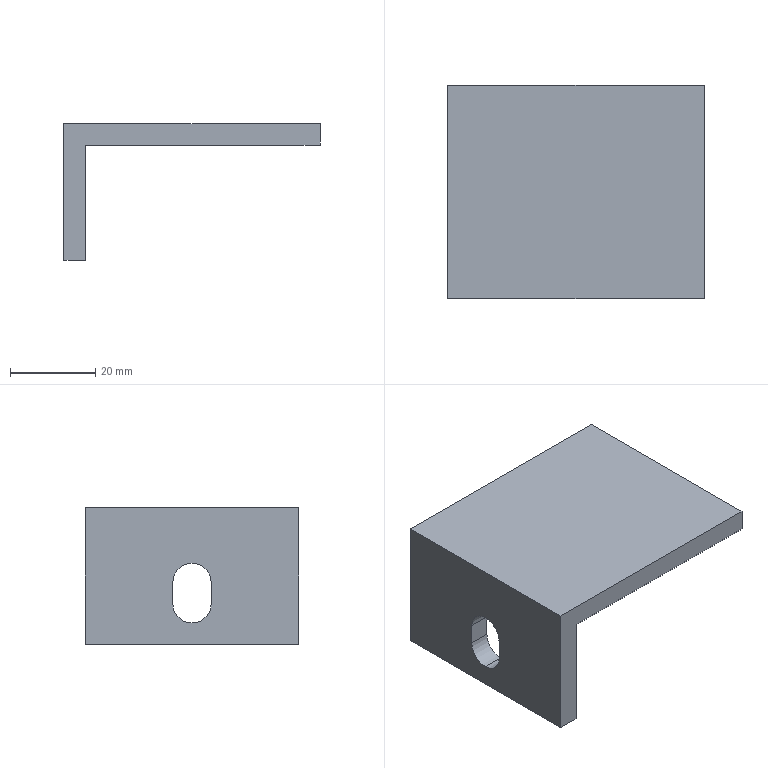Component | SolidWorks | -1-SOLID1-1 | 1 solid | 14 faces | box 60 x 50 x 32 mm | volume 21207 mm3 | plane 10 | cylinder 4 | commonest cylinder face diameters 9 x4
STEP:
#1=CARTESIAN_POINT('',(-15.551,-30.138,50.197));
#2=VERTEX_POINT('',#1);
#3=CARTESIAN_POINT('',(-15.551,-30.315,50.374));
#4=VERTEX_POINT('',#3);
#5=CARTESIAN_POINT('',(-15.551,-30.315,50.197));
#6=DIRECTION('',(1.,0.,-0.));
#7=DIRECTION('',(0.,-1.,0.));
#8=AXIS2_PLACEMENT_3D('',#5,#6,#7);
#9=CIRCLE('',#8,0.1772);
#10=EDGE_CURVE('',#2,#4,#9,.T.);
#11=ORIENTED_EDGE('',*,*,#10,.T.);
#12=CARTESIAN_POINT('',(-15.748,-30.315,50.374));
#13=VERTEX_POINT('',#12);
#14=CARTESIAN_POINT('',(-13.386,-30.315,50.374));
#15=DIRECTION('',(-1.,-0.,0.));
#16=VECTOR('',#15,39.37);
#17=LINE('',#14,#16);
#18=EDGE_CURVE('',#4,#13,#17,.T.);
#19=ORIENTED_EDGE('',*,*,#18,.T.);
#20=CARTESIAN_POINT('',(-15.748,-30.138,50.197));
#21=VERTEX_POINT('',#20);
#22=CARTESIAN_POINT('',(-15.748,-30.315,50.197));
#23=DIRECTION('',(-1.,-0.,0.));
#24=DIRECTION('',(0.,0.,1.));
#25=AXIS2_PLACEMENT_3D('',#22,#23,#24);
#26=CIRCLE('',#25,0.1772);
#27=EDGE_CURVE('',#13,#21,#26,.T.);
#28=ORIENTED_EDGE('',*,*,#27,.T.);
#29=CARTESIAN_POINT('',(-13.386,-30.138,50.197));
#30=DIRECTION('',(-1.,-0.,0.));
#31=VECTOR('',#30,39.37);
#32=LINE('',#29,#31);
#33=EDGE_CURVE('',#2,#21,#32,.T.);
#34=ORIENTED_EDGE('',*,*,#33,.F.);
#35=EDGE_LOOP('',(#11,#19,#28,#34));
#36=FACE_OUTER_BOUND('',#35,.T.);
#37=CARTESIAN_POINT('',(-13.386,-30.315,50.197));
#38=DIRECTION('',(-1.,-0.,0.));
#39=DIRECTION('',(0.,0.,1.));
#40=AXIS2_PLACEMENT_3D('',#37,#38,#39);
#41=CYLINDRICAL_SURFACE('',#40,0.1772);
#42=ADVANCED_FACE('',(#36),#41,.F.);
#43=CARTESIAN_POINT('',(-15.551,-30.492,50.));
#44=VERTEX_POINT('',#43);
#45=CARTESIAN_POINT('',(-15.551,-30.315,49.823));
#46=VERTEX_POINT('',#45);
#47=CARTESIAN_POINT('',(-15.551,-30.315,50.));
#48=DIRECTION('',(1.,0.,-0.));
#49=DIRECTION('',(0.,-1.,0.));
#50=AXIS2_PLACEMENT_3D('',#47,#48,#49);
#51=CIRCLE('',#50,0.1772);
#52=EDGE_CURVE('',#44,#46,#51,.T.);
#53=ORIENTED_EDGE('',*,*,#52,.T.);
#54=CARTESIAN_POINT('',(-15.748,-30.315,49.823));
#55=VERTEX_POINT('',#54);
#56=CARTESIAN_POINT('',(-13.386,-30.315,49.823));
#57=DIRECTION('',(-1.,-0.,0.));
#58=VECTOR('',#57,39.37);
#59=LINE('',#56,#58);
#60=EDGE_CURVE('',#46,#55,#59,.T.);
#61=ORIENTED_EDGE('',*,*,#60,.T.);
#62=CARTESIAN_POINT('',(-15.748,-30.492,50.));
#63=VERTEX_POINT('',#62);
#64=CARTESIAN_POINT('',(-15.748,-30.315,50.));
#65=DIRECTION('',(-1.,-0.,0.));
#66=DIRECTION('',(0.,0.,-1.));
#67=AXIS2_PLACEMENT_3D('',#64,#65,#66);
#68=CIRCLE('',#67,0.1772);
#69=EDGE_CURVE('',#55,#63,#68,.T.);
#70=ORIENTED_EDGE('',*,*,#69,.T.);
#71=CARTESIAN_POINT('',(-13.386,-30.492,50.));
#72=DIRECTION('',(-1.,-0.,0.));
#73=VECTOR('',#72,39.37);
#74=LINE('',#71,#73);
#75=EDGE_CURVE('',#44,#63,#74,.T.);
#76=ORIENTED_EDGE('',*,*,#75,.F.);
#77=EDGE_LOOP('',(#53,#61,#70,#76));
#78=FACE_OUTER_BOUND('',#77,.T.);
#79=CARTESIAN_POINT('',(-13.386,-30.315,50.));
#80=DIRECTION('',(-1.,-0.,0.));
#81=DIRECTION('',(0.,0.,1.));
#82=AXIS2_PLACEMENT_3D('',#79,#80,#81);
#83=CYLINDRICAL_SURFACE('',#82,0.1772);
#84=ADVANCED_FACE('',(#78),#83,.F.);
#85=CARTESIAN_POINT('',(-13.386,-29.331,50.886));
#86=VERTEX_POINT('',#85);
#87=CARTESIAN_POINT('',(-15.748,-29.331,50.886));
#88=VERTEX_POINT('',#87);
#89=CARTESIAN_POINT('',(-13.386,-29.331,50.886));
#90=DIRECTION('',(-1.,-0.,0.));
#91=VECTOR('',#90,39.37);
#92=LINE('',#89,#91);
#93=EDGE_CURVE('',#86,#88,#92,.T.);
#94=ORIENTED_EDGE('',*,*,#93,.T.);
#95=CARTESIAN_POINT('',(-15.748,-31.299,50.886));
#96=VERTEX_POINT('',#95);
#97=CARTESIAN_POINT('',(-15.748,-31.299,50.886));
#98=DIRECTION('',(-0.,1.,0.));
#99=VECTOR('',#98,39.37);
#100=LINE('',#97,#99);
#101=EDGE_CURVE('',#96,#88,#100,.T.);
#102=ORIENTED_EDGE('',*,*,#101,.F.);
#103=CARTESIAN_POINT('',(-13.386,-31.299,50.886));
#104=VERTEX_POINT('',#103);
#105=CARTESIAN_POINT('',(-13.386,-31.299,50.886));
#106=DIRECTION('',(-1.,-0.,0.));
#107=VECTOR('',#106,39.37);
#108=LINE('',#105,#107);
#109=EDGE_CURVE('',#104,#96,#108,.T.);
#110=ORIENTED_EDGE('',*,*,#109,.F.);
#111=CARTESIAN_POINT('',(-13.386,-31.299,50.886));
#112=DIRECTION('',(-0.,1.,0.));
#113=VECTOR('',#112,39.37);
#114=LINE('',#111,#113);
#115=EDGE_CURVE('',#104,#86,#114,.T.);
#116=ORIENTED_EDGE('',*,*,#115,.T.);
#117=EDGE_LOOP('',(#94,#102,#110,#116));
#118=FACE_OUTER_BOUND('',#117,.T.);
#119=CARTESIAN_POINT('',(-13.386,-31.299,50.886));
#120=DIRECTION('',(-0.,-0.,-1.));
#121=DIRECTION('',(0.,-1.,0.));
#122=AXIS2_PLACEMENT_3D('',#119,#120,#121);
#123=PLANE('',#122);
#124=ADVANCED_FACE('',(#118),#123,.F.);
#125=CARTESIAN_POINT('',(-15.748,-30.492,50.197));
#126=VERTEX_POINT('',#125);
#127=CARTESIAN_POINT('',(-15.748,-30.492,50.197));
#128=DIRECTION('',(-0.,-0.,1.));
#129=VECTOR('',#128,39.37);
#130=LINE('',#127,#129);
#131=EDGE_CURVE('',#63,#126,#130,.T.);
#132=ORIENTED_EDGE('',*,*,#131,.F.);
#133=ORIENTED_EDGE('',*,*,#69,.F.);
#134=CARTESIAN_POINT('',(-15.748,-30.138,50.));
#135=VERTEX_POINT('',#134);
#136=CARTESIAN_POINT('',(-15.748,-30.315,50.));
#137=DIRECTION('',(-1.,-0.,0.));
#138=DIRECTION('',(0.,0.,-1.));
#139=AXIS2_PLACEMENT_3D('',#136,#137,#138);
#140=CIRCLE('',#139,0.1772);
#141=EDGE_CURVE('',#135,#55,#140,.T.);
#142=ORIENTED_EDGE('',*,*,#141,.F.);
#143=CARTESIAN_POINT('',(-15.748,-30.138,50.197));
#144=DIRECTION('',(0.,0.,-1.));
#145=VECTOR('',#144,39.37);
#146=LINE('',#143,#145);
#147=EDGE_CURVE('',#21,#135,#146,.T.);
#148=ORIENTED_EDGE('',*,*,#147,.F.);
#149=ORIENTED_EDGE('',*,*,#27,.F.);
#150=CARTESIAN_POINT('',(-15.748,-30.315,50.197));
#151=DIRECTION('',(-1.,-0.,0.));
#152=DIRECTION('',(0.,0.,1.));
#153=AXIS2_PLACEMENT_3D('',#150,#151,#152);
#154=CIRCLE('',#153,0.1772);
#155=EDGE_CURVE('',#126,#13,#154,.T.);
#156=ORIENTED_EDGE('',*,*,#155,.F.);
#157=EDGE_LOOP('',(#132,#133,#142,#148,#149,#156));
#158=FACE_BOUND('',#157,.T.);
#159=CARTESIAN_POINT('',(-15.748,-29.331,49.626));
#160=VERTEX_POINT('',#159);
#161=CARTESIAN_POINT('',(-15.748,-29.331,50.886));
#162=DIRECTION('',(0.,0.,-1.));
#163=VECTOR('',#162,39.37);
#164=LINE('',#161,#163);
#165=EDGE_CURVE('',#88,#160,#164,.T.);
#166=ORIENTED_EDGE('',*,*,#165,.T.);
#167=CARTESIAN_POINT('',(-15.748,-31.299,49.626));
#168=VERTEX_POINT('',#167);
#169=CARTESIAN_POINT('',(-15.748,-31.299,49.626));
#170=DIRECTION('',(-0.,1.,0.));
#171=VECTOR('',#170,39.37);
#172=LINE('',#169,#171);
#173=EDGE_CURVE('',#168,#160,#172,.T.);
#174=ORIENTED_EDGE('',*,*,#173,.F.);
#175=CARTESIAN_POINT('',(-15.748,-31.299,50.886));
#176=DIRECTION('',(0.,0.,-1.));
#177=VECTOR('',#176,39.37);
#178=LINE('',#175,#177);
#179=EDGE_CURVE('',#96,#168,#178,.T.);
#180=ORIENTED_EDGE('',*,*,#179,.F.);
#181=ORIENTED_EDGE('',*,*,#101,.T.);
#182=EDGE_LOOP('',(#166,#174,#180,#181));
#183=FACE_OUTER_BOUND('',#182,.T.);
#184=CARTESIAN_POINT('',(-15.748,-31.299,50.886));
#185=DIRECTION('',(1.,0.,0.));
#186=DIRECTION('',(0.,0.,-1.));
#187=AXIS2_PLACEMENT_3D('',#184,#185,#186);
#188=PLANE('',#187);
#189=ADVANCED_FACE('',(#158,#183),#188,.F.);
#190=CARTESIAN_POINT('',(-15.551,-29.331,49.626));
#191=VERTEX_POINT('',#190);
#192=CARTESIAN_POINT('',(-15.748,-29.331,49.626));
#193=DIRECTION('',(1.,0.,-0.));
#194=VECTOR('',#193,39.37);
#195=LINE('',#192,#194);
#196=EDGE_CURVE('',#160,#191,#195,.T.);
#197=ORIENTED_EDGE('',*,*,#196,.T.);
#198=CARTESIAN_POINT('',(-15.551,-31.299,49.626));
#199=VERTEX_POINT('',#198);
#200=CARTESIAN_POINT('',(-15.551,-31.299,49.626));
#201=DIRECTION('',(-0.,1.,0.));
#202=VECTOR('',#201,39.37);
#203=LINE('',#200,#202);
#204=EDGE_CURVE('',#199,#191,#203,.T.);
#205=ORIENTED_EDGE('',*,*,#204,.F.);
#206=CARTESIAN_POINT('',(-15.748,-31.299,49.626));
#207=DIRECTION('',(1.,0.,-0.));
#208=VECTOR('',#207,39.37);
#209=LINE('',#206,#208);
#210=EDGE_CURVE('',#168,#199,#209,.T.);
#211=ORIENTED_EDGE('',*,*,#210,.F.);
#212=ORIENTED_EDGE('',*,*,#173,.T.);
#213=EDGE_LOOP('',(#197,#205,#211,#212));
#214=FACE_OUTER_BOUND('',#213,.T.);
#215=CARTESIAN_POINT('',(-15.748,-31.299,49.626));
#216=DIRECTION('',(0.,0.,1.));
#217=DIRECTION('',(-0.,1.,0.));
#218=AXIS2_PLACEMENT_3D('',#215,#216,#217);
#219=PLANE('',#218);
#220=ADVANCED_FACE('',(#214),#219,.F.);
#221=CARTESIAN_POINT('',(-15.551,-30.138,50.));
#222=VERTEX_POINT('',#221);
#223=CARTESIAN_POINT('',(-15.551,-30.138,50.197));
#224=DIRECTION('',(0.,0.,1.));
#225=VECTOR('',#224,39.37);
#226=LINE('',#223,#225);
#227=EDGE_CURVE('',#222,#2,#226,.T.);
#228=ORIENTED_EDGE('',*,*,#227,.F.);
#229=CARTESIAN_POINT('',(-15.551,-30.315,50.));
#230=DIRECTION('',(1.,0.,-0.));
#231=DIRECTION('',(0.,-1.,0.));
#232=AXIS2_PLACEMENT_3D('',#229,#230,#231);
#233=CIRCLE('',#232,0.1772);
#234=EDGE_CURVE('',#46,#222,#233,.T.);
#235=ORIENTED_EDGE('',*,*,#234,.F.);
#236=ORIENTED_EDGE('',*,*,#52,.F.);
#237=CARTESIAN_POINT('',(-15.551,-30.492,50.197));
#238=VERTEX_POINT('',#237);
#239=CARTESIAN_POINT('',(-15.551,-30.492,50.197));
#240=DIRECTION('',(-0.,-0.,-1.));
#241=VECTOR('',#240,39.37);
#242=LINE('',#239,#241);
#243=EDGE_CURVE('',#238,#44,#242,.T.);
#244=ORIENTED_EDGE('',*,*,#243,.F.);
#245=CARTESIAN_POINT('',(-15.551,-30.315,50.197));
#246=DIRECTION('',(1.,0.,-0.));
#247=DIRECTION('',(0.,-1.,0.));
#248=AXIS2_PLACEMENT_3D('',#245,#246,#247);
#249=CIRCLE('',#248,0.1772);
#250=EDGE_CURVE('',#4,#238,#249,.T.);
#251=ORIENTED_EDGE('',*,*,#250,.F.);
#252=ORIENTED_EDGE('',*,*,#10,.F.);
#253=EDGE_LOOP('',(#228,#235,#236,#244,#251,#252));
#254=FACE_BOUND('',#253,.T.);
#255=CARTESIAN_POINT('',(-15.551,-29.331,50.689));
#256=VERTEX_POINT('',#255);
#257=CARTESIAN_POINT('',(-15.551,-29.331,49.626));
#258=DIRECTION('',(0.,0.,1.));
#259=VECTOR('',#258,39.37);
#260=LINE('',#257,#259);
#261=EDGE_CURVE('',#191,#256,#260,.T.);
#262=ORIENTED_EDGE('',*,*,#261,.T.);
#263=CARTESIAN_POINT('',(-15.551,-31.299,50.689));
#264=VERTEX_POINT('',#263);
#265=CARTESIAN_POINT('',(-15.551,-31.299,50.689));
#266=DIRECTION('',(-0.,1.,0.));
#267=VECTOR('',#266,39.37);
#268=LINE('',#265,#267);
#269=EDGE_CURVE('',#264,#256,#268,.T.);
#270=ORIENTED_EDGE('',*,*,#269,.F.);
#271=CARTESIAN_POINT('',(-15.551,-31.299,49.626));
#272=DIRECTION('',(0.,0.,1.));
#273=VECTOR('',#272,39.37);
#274=LINE('',#271,#273);
#275=EDGE_CURVE('',#199,#264,#274,.T.);
#276=ORIENTED_EDGE('',*,*,#275,.F.);
#277=ORIENTED_EDGE('',*,*,#204,.T.);
#278=EDGE_LOOP('',(#262,#270,#276,#277));
#279=FACE_OUTER_BOUND('',#278,.T.);
#280=CARTESIAN_POINT('',(-15.551,-31.299,49.626));
#281=DIRECTION('',(-1.,-0.,0.));
#282=DIRECTION('',(-0.,1.,0.));
#283=AXIS2_PLACEMENT_3D('',#280,#281,#282);
#284=PLANE('',#283);
#285=ADVANCED_FACE('',(#254,#279),#284,.F.);
#286=CARTESIAN_POINT('',(-13.386,-29.331,50.689));
#287=VERTEX_POINT('',#286);
#288=CARTESIAN_POINT('',(-15.551,-29.331,50.689));
#289=DIRECTION('',(1.,0.,-0.));
#290=VECTOR('',#289,39.37);
#291=LINE('',#288,#290);
#292=EDGE_CURVE('',#256,#287,#291,.T.);
#293=ORIENTED_EDGE('',*,*,#292,.T.);
#294=CARTESIAN_POINT('',(-13.386,-31.299,50.689));
#295=VERTEX_POINT('',#294);
#296=CARTESIAN_POINT('',(-13.386,-31.299,50.689));
#297=DIRECTION('',(-0.,1.,0.));
#298=VECTOR('',#297,39.37);
#299=LINE('',#296,#298);
#300=EDGE_CURVE('',#295,#287,#299,.T.);
#301=ORIENTED_EDGE('',*,*,#300,.F.);
#302=CARTESIAN_POINT('',(-15.551,-31.299,50.689));
#303=DIRECTION('',(1.,0.,-0.));
#304=VECTOR('',#303,39.37);
#305=LINE('',#302,#304);
#306=EDGE_CURVE('',#264,#295,#305,.T.);
#307=ORIENTED_EDGE('',*,*,#306,.F.);
#308=ORIENTED_EDGE('',*,*,#269,.T.);
#309=EDGE_LOOP('',(#293,#301,#307,#308));
#310=FACE_OUTER_BOUND('',#309,.T.);
#311=CARTESIAN_POINT('',(-15.551,-31.299,50.689));
#312=DIRECTION('',(0.,0.,1.));
#313=DIRECTION('',(-0.,1.,0.));
#314=AXIS2_PLACEMENT_3D('',#311,#312,#313);
#315=PLANE('',#314);
#316=ADVANCED_FACE('',(#310),#315,.F.);
#317=CARTESIAN_POINT('',(-13.386,-29.331,50.689));
#318=DIRECTION('',(0.,0.,1.));
#319=VECTOR('',#318,39.37);
#320=LINE('',#317,#319);
#321=EDGE_CURVE('',#287,#86,#320,.T.);
#322=ORIENTED_EDGE('',*,*,#321,.T.);
#323=ORIENTED_EDGE('',*,*,#115,.F.);
#324=CARTESIAN_POINT('',(-13.386,-31.299,50.689));
#325=DIRECTION('',(0.,0.,1.));
#326=VECTOR('',#325,39.37);
#327=LINE('',#324,#326);
#328=EDGE_CURVE('',#295,#104,#327,.T.);
#329=ORIENTED_EDGE('',*,*,#328,.F.);
#330=ORIENTED_EDGE('',*,*,#300,.T.);
#331=EDGE_LOOP('',(#322,#323,#329,#330));
#332=FACE_OUTER_BOUND('',#331,.T.);
#333=CARTESIAN_POINT('',(-13.386,-31.299,50.689));
#334=DIRECTION('',(-1.,-0.,0.));
#335=DIRECTION('',(-0.,1.,0.));
#336=AXIS2_PLACEMENT_3D('',#333,#334,#335);
#337=PLANE('',#336);
#338=ADVANCED_FACE('',(#332),#337,.F.);
#339=ORIENTED_EDGE('',*,*,#109,.T.);
#340=ORIENTED_EDGE('',*,*,#179,.T.);
#341=ORIENTED_EDGE('',*,*,#210,.T.);
#342=ORIENTED_EDGE('',*,*,#275,.T.);
#343=ORIENTED_EDGE('',*,*,#306,.T.);
#344=ORIENTED_EDGE('',*,*,#328,.T.);
#345=EDGE_LOOP('',(#339,#340,#341,#342,#343,#344));
#346=FACE_OUTER_BOUND('',#345,.T.);
#347=CARTESIAN_POINT('',(-15.748,-31.299,50.886));
#348=DIRECTION('',(0.,-1.,-0.));
#349=DIRECTION('',(-1.,-0.,0.));
#350=AXIS2_PLACEMENT_3D('',#347,#348,#349);
#351=PLANE('',#350);
#352=ADVANCED_FACE('',(#346),#351,.T.);
#353=ORIENTED_EDGE('',*,*,#93,.F.);
#354=ORIENTED_EDGE('',*,*,#321,.F.);
#355=ORIENTED_EDGE('',*,*,#292,.F.);
#356=ORIENTED_EDGE('',*,*,#261,.F.);
#357=ORIENTED_EDGE('',*,*,#196,.F.);
#358=ORIENTED_EDGE('',*,*,#165,.F.);
#359=EDGE_LOOP('',(#353,#354,#355,#356,#357,#358));
#360=FACE_OUTER_BOUND('',#359,.T.);
#361=CARTESIAN_POINT('',(-15.748,-29.331,50.886));
#362=DIRECTION('',(0.,-1.,-0.));
#363=DIRECTION('',(-1.,-0.,0.));
#364=AXIS2_PLACEMENT_3D('',#361,#362,#363);
#365=PLANE('',#364);
#366=ADVANCED_FACE('',(#360),#365,.F.);
#367=ORIENTED_EDGE('',*,*,#60,.F.);
#368=ORIENTED_EDGE('',*,*,#234,.T.);
#369=CARTESIAN_POINT('',(-13.386,-30.138,50.));
#370=DIRECTION('',(-1.,-0.,0.));
#371=VECTOR('',#370,39.37);
#372=LINE('',#369,#371);
#373=EDGE_CURVE('',#222,#135,#372,.T.);
#374=ORIENTED_EDGE('',*,*,#373,.T.);
#375=ORIENTED_EDGE('',*,*,#141,.T.);
#376=EDGE_LOOP('',(#367,#368,#374,#375));
#377=FACE_OUTER_BOUND('',#376,.T.);
#378=CARTESIAN_POINT('',(-13.386,-30.315,50.));
#379=DIRECTION('',(-1.,-0.,0.));
#380=DIRECTION('',(0.,0.,1.));
#381=AXIS2_PLACEMENT_3D('',#378,#379,#380);
#382=CYLINDRICAL_SURFACE('',#381,0.1772);
#383=ADVANCED_FACE('',(#377),#382,.F.);
#384=ORIENTED_EDGE('',*,*,#227,.T.);
#385=ORIENTED_EDGE('',*,*,#33,.T.);
#386=ORIENTED_EDGE('',*,*,#147,.T.);
#387=ORIENTED_EDGE('',*,*,#373,.F.);
#388=EDGE_LOOP('',(#384,#385,#386,#387));
#389=FACE_OUTER_BOUND('',#388,.T.);
#390=CARTESIAN_POINT('',(-13.386,-30.138,50.197));
#391=DIRECTION('',(-0.,1.,0.));
#392=DIRECTION('',(1.,0.,-0.));
#393=AXIS2_PLACEMENT_3D('',#390,#391,#392);
#394=PLANE('',#393);
#395=ADVANCED_FACE('',(#389),#394,.F.);
#396=ORIENTED_EDGE('',*,*,#18,.F.);
#397=ORIENTED_EDGE('',*,*,#250,.T.);
#398=CARTESIAN_POINT('',(-13.386,-30.492,50.197));
#399=DIRECTION('',(-1.,-0.,0.));
#400=VECTOR('',#399,39.37);
#401=LINE('',#398,#400);
#402=EDGE_CURVE('',#238,#126,#401,.T.);
#403=ORIENTED_EDGE('',*,*,#402,.T.);
#404=ORIENTED_EDGE('',*,*,#155,.T.);
#405=EDGE_LOOP('',(#396,#397,#403,#404));
#406=FACE_OUTER_BOUND('',#405,.T.);
#407=CARTESIAN_POINT('',(-13.386,-30.315,50.197));
#408=DIRECTION('',(-1.,-0.,0.));
#409=DIRECTION('',(0.,0.,1.));
#410=AXIS2_PLACEMENT_3D('',#407,#408,#409);
#411=CYLINDRICAL_SURFACE('',#410,0.1772);
#412=ADVANCED_FACE('',(#406),#411,.F.);
#413=ORIENTED_EDGE('',*,*,#243,.T.);
#414=ORIENTED_EDGE('',*,*,#75,.T.);
#415=ORIENTED_EDGE('',*,*,#131,.T.);
#416=ORIENTED_EDGE('',*,*,#402,.F.);
#417=EDGE_LOOP('',(#413,#414,#415,#416));
#418=FACE_OUTER_BOUND('',#417,.T.);
#419=CARTESIAN_POINT('',(-13.386,-30.492,50.197));
#420=DIRECTION('',(0.,-1.,-0.));
#421=DIRECTION('',(-1.,-0.,0.));
#422=AXIS2_PLACEMENT_3D('',#419,#420,#421);
#423=PLANE('',#422);
#424=ADVANCED_FACE('',(#418),#423,.F.);
#425=CLOSED_SHELL('',(#42,#84,#124,#189,#220,#285,#316,#338,#352,#366,#383,#395,#412,#424));
#426=MANIFOLD_SOLID_BREP('',#425);
#427=CARTESIAN_POINT('',(0.,0.,0.));
#428=DIRECTION('',(0.,0.,1.));
#429=DIRECTION('',(1.,0.,0.));
#430=AXIS2_PLACEMENT_3D('',#427,#428,#429);
#431=(LENGTH_UNIT()NAMED_UNIT(*)SI_UNIT($,.METRE.));
#432=LENGTH_MEASURE_WITH_UNIT(LENGTH_MEASURE(0.0254),#431);
#433=DIMENSIONAL_EXPONENTS(1.,0.,0.,0.,0.,0.,0.);
#434=(CONVERSION_BASED_UNIT('',#432)LENGTH_UNIT()NAMED_UNIT(#433));
#435=UNCERTAINTY_MEASURE_WITH_UNIT(LENGTH_MEASURE(0.00001),#434,'','');
#436=(NAMED_UNIT(*)PLANE_ANGLE_UNIT()SI_UNIT($,.RADIAN.));
#437=(NAMED_UNIT(*)SI_UNIT($,.STERADIAN.)SOLID_ANGLE_UNIT());
#438=(GEOMETRIC_REPRESENTATION_CONTEXT(3)GLOBAL_UNCERTAINTY_ASSIGNED_CONTEXT((#435))GLOBAL_UNIT_ASSIGNED_CONTEXT((#434,#436,#437))REPRESENTATION_CONTEXT('',''));
#439=ADVANCED_BREP_SHAPE_REPRESENTATION('',(#426,#430),#438);
#440=COLOUR_RGB('',0.7922,0.8196,0.9333);
#441=FILL_AREA_STYLE_COLOUR('',#440);
#442=FILL_AREA_STYLE('',(#441));
#443=SURFACE_STYLE_FILL_AREA(#442);
#444=SURFACE_SIDE_STYLE('',(#443));
#445=SURFACE_STYLE_USAGE(.BOTH.,#444);
#446=PRESENTATION_STYLE_ASSIGNMENT((#445));
#447=STYLED_ITEM('',(#446),#426);
#448=(LENGTH_UNIT()NAMED_UNIT(*)SI_UNIT($,.METRE.));
#449=LENGTH_MEASURE_WITH_UNIT(LENGTH_MEASURE(0.0254),#448);
#450=DIMENSIONAL_EXPONENTS(1.,0.,0.,0.,0.,0.,0.);
#451=(CONVERSION_BASED_UNIT('',#449)LENGTH_UNIT()NAMED_UNIT(#450));
#452=UNCERTAINTY_MEASURE_WITH_UNIT(LENGTH_MEASURE(0.00001),#451,'','');
#453=(NAMED_UNIT(*)PLANE_ANGLE_UNIT()SI_UNIT($,.RADIAN.));
#454=(NAMED_UNIT(*)SI_UNIT($,.STERADIAN.)SOLID_ANGLE_UNIT());
#455=(GEOMETRIC_REPRESENTATION_CONTEXT(3)GLOBAL_UNCERTAINTY_ASSIGNED_CONTEXT((#452))GLOBAL_UNIT_ASSIGNED_CONTEXT((#451,#453,#454))REPRESENTATION_CONTEXT('',''));
#456=MECHANICAL_DESIGN_GEOMETRIC_PRESENTATION_REPRESENTATION('',(#447),#455);
#457=PRESENTATION_LAYER_ASSIGNMENT('','',(#447));